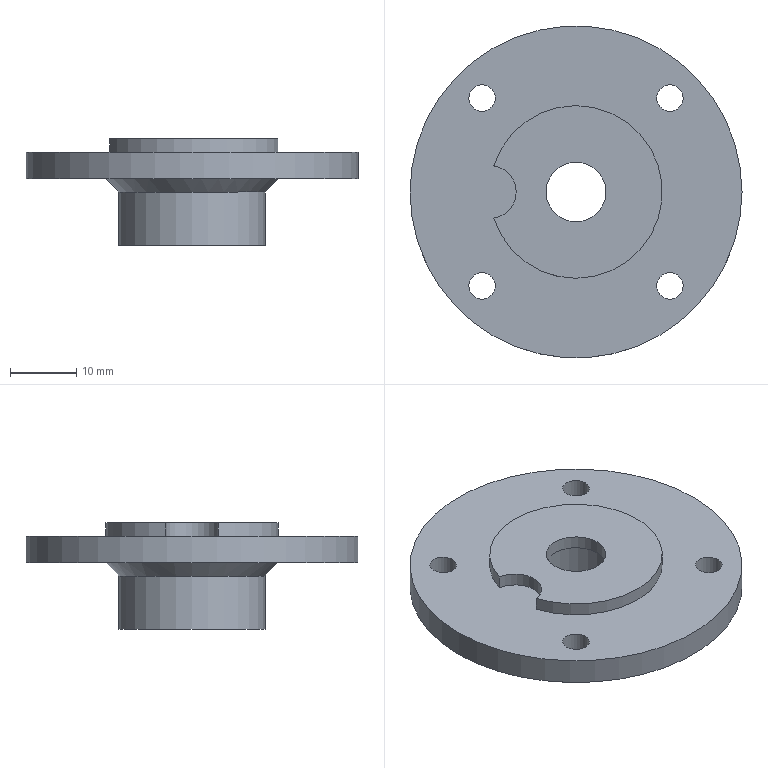Component | NX | 07__27_2 | 1 solid | 16 faces | box 50 x 50 x 16 mm | volume 10905 mm3 | cylinder 10 | plane 5 | cone 1 | commonest cylinder face diameters 4 x4 9 x1 12 x1 22 x1 50 x1 26 x1 8 x1
STEP:
#1=CARTESIAN_POINT('',(0.,0.,0.));
#2=DIRECTION('',(0.,0.,1.));
#3=DIRECTION('',(1.,0.,0.));
#4=AXIS2_PLACEMENT_3D('',#1,#2,#3);
#5=CARTESIAN_POINT('',(111.522,109.608,186.432));
#6=VERTEX_POINT('',#5);
#7=CARTESIAN_POINT('',(116.022,109.608,186.432));
#8=DIRECTION('',(0.,0.,-1.));
#9=DIRECTION('',(-1.,0.,-0.));
#10=AXIS2_PLACEMENT_3D('',#7,#8,#9);
#11=CIRCLE('',#10,4.5);
#12=CARTESIAN_POINT('',(116.022,109.608,188.432));
#13=DIRECTION('',(0.,0.,-1.));
#14=DIRECTION('',(-1.,0.,-0.));
#15=AXIS2_PLACEMENT_3D('',#12,#13,#14);
#16=CYLINDRICAL_SURFACE('',#15,4.5);
#17=CARTESIAN_POINT('',(0.,2.));
#18=DIRECTION('',(1.,0.));
#19=VECTOR('',#18,1.);
#20=LINE('',#17,#19);
#21=(GEOMETRIC_REPRESENTATION_CONTEXT(2)PARAMETRIC_REPRESENTATION_CONTEXT()REPRESENTATION_CONTEXT('',''));
#22=DEFINITIONAL_REPRESENTATION('',(#20),#21);
#23=PCURVE('',#16,#22);
#24=CARTESIAN_POINT('',(111.522,109.608,186.432));
#25=DIRECTION('',(0.,0.,-1.));
#26=DIRECTION('',(-1.,0.,-0.));
#27=AXIS2_PLACEMENT_3D('',#24,#25,#26);
#28=PLANE('',#27);
#29=CARTESIAN_POINT('',(-4.5,0.));
#30=DIRECTION('',(1.,0.));
#31=AXIS2_PLACEMENT_2D('',#29,#30);
#32=CIRCLE('',#31,4.5);
#33=(GEOMETRIC_REPRESENTATION_CONTEXT(2)PARAMETRIC_REPRESENTATION_CONTEXT()REPRESENTATION_CONTEXT('',''));
#34=DEFINITIONAL_REPRESENTATION('',(#32),#33);
#35=PCURVE('',#28,#34);
#36=SURFACE_CURVE('',#11,(#23,#35),.PCURVE_S1.);
#37=EDGE_CURVE('',#6,#6,#36,.T.);
#38=ORIENTED_EDGE('',*,*,#37,.F.);
#39=CARTESIAN_POINT('',(111.522,109.608,188.432));
#40=VERTEX_POINT('',#39);
#41=CARTESIAN_POINT('',(111.522,109.608,188.432));
#42=CARTESIAN_POINT('',(111.522,109.608,186.432));
#43=B_SPLINE_CURVE_WITH_KNOTS('',1,(#41,#42),.UNSPECIFIED.,.F.,.F.,(2,2),(0.,2.),.PIECEWISE_BEZIER_KNOTS.);
#44=CARTESIAN_POINT('',(0.,0.));
#45=DIRECTION('',(0.,1.));
#46=VECTOR('',#45,1.);
#47=LINE('',#44,#46);
#48=(GEOMETRIC_REPRESENTATION_CONTEXT(2)PARAMETRIC_REPRESENTATION_CONTEXT()REPRESENTATION_CONTEXT('',''));
#49=DEFINITIONAL_REPRESENTATION('',(#47),#48);
#50=PCURVE('',#16,#49);
#51=CARTESIAN_POINT('',(6.283,0.));
#52=DIRECTION('',(0.,1.));
#53=VECTOR('',#52,1.);
#54=LINE('',#51,#53);
#55=(GEOMETRIC_REPRESENTATION_CONTEXT(2)PARAMETRIC_REPRESENTATION_CONTEXT()REPRESENTATION_CONTEXT('',''));
#56=DEFINITIONAL_REPRESENTATION('',(#54),#55);
#57=PCURVE('',#16,#56);
#58=SEAM_CURVE('',#43,(#50,#57),.PCURVE_S1.);
#59=EDGE_CURVE('',#40,#6,#58,.T.);
#60=ORIENTED_EDGE('',*,*,#59,.F.);
#61=CARTESIAN_POINT('',(116.022,109.608,188.432));
#62=DIRECTION('',(0.,0.,-1.));
#63=DIRECTION('',(-1.,0.,-0.));
#64=AXIS2_PLACEMENT_3D('',#61,#62,#63);
#65=CIRCLE('',#64,4.5);
#66=CARTESIAN_POINT('',(0.,0.));
#67=DIRECTION('',(1.,0.));
#68=VECTOR('',#67,1.);
#69=LINE('',#66,#68);
#70=(GEOMETRIC_REPRESENTATION_CONTEXT(2)PARAMETRIC_REPRESENTATION_CONTEXT()REPRESENTATION_CONTEXT('',''));
#71=DEFINITIONAL_REPRESENTATION('',(#69),#70);
#72=PCURVE('',#16,#71);
#73=CARTESIAN_POINT('',(103.022,109.608,188.432));
#74=DIRECTION('',(-0.,0.,1.));
#75=DIRECTION('',(1.,0.,0.));
#76=AXIS2_PLACEMENT_3D('',#73,#74,#75);
#77=PLANE('',#76);
#78=CARTESIAN_POINT('',(8.5,0.));
#79=CARTESIAN_POINT('',(8.5,7.794));
#80=CARTESIAN_POINT('',(15.25,3.897));
#81=CARTESIAN_POINT('',(22.,0.));
#82=CARTESIAN_POINT('',(15.25,-3.897));
#83=CARTESIAN_POINT('',(8.5,-7.794));
#84=CARTESIAN_POINT('',(8.5,0.));
#85=(BOUNDED_CURVE()B_SPLINE_CURVE(2,(#78,#79,#80,#81,#82,#83,#84),.UNSPECIFIED.,.T.,.F.)B_SPLINE_CURVE_WITH_KNOTS((1,2,2,2,2,1),(-2.094,0.,2.094,4.189,6.283,8.378),.UNSPECIFIED.)CURVE()GEOMETRIC_REPRESENTATION_ITEM()RATIONAL_B_SPLINE_CURVE((1.,0.5,1.,0.5,1.,0.5,1.))REPRESENTATION_ITEM(''));
#86=(GEOMETRIC_REPRESENTATION_CONTEXT(2)PARAMETRIC_REPRESENTATION_CONTEXT()REPRESENTATION_CONTEXT('',''));
#87=DEFINITIONAL_REPRESENTATION('',(#85),#86);
#88=PCURVE('',#77,#87);
#89=SURFACE_CURVE('',#65,(#72,#88),.PCURVE_S1.);
#90=EDGE_CURVE('',#40,#40,#89,.T.);
#91=ORIENTED_EDGE('',*,*,#90,.T.);
#92=ORIENTED_EDGE('',*,*,#59,.T.);
#93=EDGE_LOOP('',(#38,#60,#91,#92));
#94=FACE_BOUND('',#93,.F.);
#95=ADVANCED_FACE('',(#94),#16,.F.);
#96=CARTESIAN_POINT('',(110.022,109.608,186.432));
#97=VERTEX_POINT('',#96);
#98=CARTESIAN_POINT('',(116.022,109.608,186.432));
#99=DIRECTION('',(0.,0.,-1.));
#100=DIRECTION('',(-1.,0.,-0.));
#101=AXIS2_PLACEMENT_3D('',#98,#99,#100);
#102=CIRCLE('',#101,6.);
#103=CARTESIAN_POINT('',(-4.5,0.));
#104=DIRECTION('',(1.,0.));
#105=AXIS2_PLACEMENT_2D('',#103,#104);
#106=CIRCLE('',#105,6.);
#107=(GEOMETRIC_REPRESENTATION_CONTEXT(2)PARAMETRIC_REPRESENTATION_CONTEXT()REPRESENTATION_CONTEXT('',''));
#108=DEFINITIONAL_REPRESENTATION('',(#106),#107);
#109=PCURVE('',#28,#108);
#110=CARTESIAN_POINT('',(116.022,109.608,188.432));
#111=DIRECTION('',(0.,0.,-1.));
#112=DIRECTION('',(-1.,0.,-0.));
#113=AXIS2_PLACEMENT_3D('',#110,#111,#112);
#114=CYLINDRICAL_SURFACE('',#113,6.);
#115=CARTESIAN_POINT('',(0.,2.));
#116=DIRECTION('',(1.,0.));
#117=VECTOR('',#116,1.);
#118=LINE('',#115,#117);
#119=(GEOMETRIC_REPRESENTATION_CONTEXT(2)PARAMETRIC_REPRESENTATION_CONTEXT()REPRESENTATION_CONTEXT('',''));
#120=DEFINITIONAL_REPRESENTATION('',(#118),#119);
#121=PCURVE('',#114,#120);
#122=SURFACE_CURVE('',#102,(#109,#121),.PCURVE_S1.);
#123=EDGE_CURVE('',#97,#97,#122,.T.);
#124=ORIENTED_EDGE('',*,*,#123,.T.);
#125=EDGE_LOOP('',(#124));
#126=FACE_BOUND('',#125,.T.);
#127=ORIENTED_EDGE('',*,*,#37,.F.);
#128=EDGE_LOOP('',(#127));
#129=FACE_BOUND('',#128,.T.);
#130=ADVANCED_FACE('',(#126,#129),#28,.T.);
#131=CARTESIAN_POINT('',(110.022,109.608,172.432));
#132=VERTEX_POINT('',#131);
#133=CARTESIAN_POINT('',(116.022,109.608,172.432));
#134=DIRECTION('',(0.,0.,-1.));
#135=DIRECTION('',(-1.,0.,-0.));
#136=AXIS2_PLACEMENT_3D('',#133,#134,#135);
#137=CIRCLE('',#136,6.);
#138=CARTESIAN_POINT('',(0.,16.));
#139=DIRECTION('',(1.,0.));
#140=VECTOR('',#139,1.);
#141=LINE('',#138,#140);
#142=(GEOMETRIC_REPRESENTATION_CONTEXT(2)PARAMETRIC_REPRESENTATION_CONTEXT()REPRESENTATION_CONTEXT('',''));
#143=DEFINITIONAL_REPRESENTATION('',(#141),#142);
#144=PCURVE('',#114,#143);
#145=CARTESIAN_POINT('',(110.022,109.608,172.432));
#146=DIRECTION('',(0.,0.,-1.));
#147=DIRECTION('',(-1.,0.,-0.));
#148=AXIS2_PLACEMENT_3D('',#145,#146,#147);
#149=PLANE('',#148);
#150=CARTESIAN_POINT('',(-6.,0.));
#151=DIRECTION('',(1.,0.));
#152=AXIS2_PLACEMENT_2D('',#150,#151);
#153=CIRCLE('',#152,6.);
#154=(GEOMETRIC_REPRESENTATION_CONTEXT(2)PARAMETRIC_REPRESENTATION_CONTEXT()REPRESENTATION_CONTEXT('',''));
#155=DEFINITIONAL_REPRESENTATION('',(#153),#154);
#156=PCURVE('',#149,#155);
#157=SURFACE_CURVE('',#137,(#144,#156),.PCURVE_S1.);
#158=EDGE_CURVE('',#132,#132,#157,.T.);
#159=ORIENTED_EDGE('',*,*,#158,.F.);
#160=CARTESIAN_POINT('',(110.022,109.608,186.432));
#161=CARTESIAN_POINT('',(110.022,109.608,172.432));
#162=B_SPLINE_CURVE_WITH_KNOTS('',1,(#160,#161),.UNSPECIFIED.,.F.,.F.,(2,2),(2.,16.),.PIECEWISE_BEZIER_KNOTS.);
#163=CARTESIAN_POINT('',(0.,0.));
#164=DIRECTION('',(0.,1.));
#165=VECTOR('',#164,1.);
#166=LINE('',#163,#165);
#167=(GEOMETRIC_REPRESENTATION_CONTEXT(2)PARAMETRIC_REPRESENTATION_CONTEXT()REPRESENTATION_CONTEXT('',''));
#168=DEFINITIONAL_REPRESENTATION('',(#166),#167);
#169=PCURVE('',#114,#168);
#170=CARTESIAN_POINT('',(6.283,0.));
#171=DIRECTION('',(0.,1.));
#172=VECTOR('',#171,1.);
#173=LINE('',#170,#172);
#174=(GEOMETRIC_REPRESENTATION_CONTEXT(2)PARAMETRIC_REPRESENTATION_CONTEXT()REPRESENTATION_CONTEXT('',''));
#175=DEFINITIONAL_REPRESENTATION('',(#173),#174);
#176=PCURVE('',#114,#175);
#177=SEAM_CURVE('',#162,(#169,#176),.PCURVE_S1.);
#178=EDGE_CURVE('',#97,#132,#177,.T.);
#179=ORIENTED_EDGE('',*,*,#178,.F.);
#180=ORIENTED_EDGE('',*,*,#123,.T.);
#181=ORIENTED_EDGE('',*,*,#178,.T.);
#182=EDGE_LOOP('',(#159,#179,#180,#181));
#183=FACE_BOUND('',#182,.F.);
#184=ADVANCED_FACE('',(#183),#114,.F.);
#185=CARTESIAN_POINT('',(105.022,109.608,172.432));
#186=VERTEX_POINT('',#185);
#187=CARTESIAN_POINT('',(116.022,109.608,172.432));
#188=DIRECTION('',(0.,0.,-1.));
#189=DIRECTION('',(-1.,0.,-0.));
#190=AXIS2_PLACEMENT_3D('',#187,#188,#189);
#191=CIRCLE('',#190,11.);
#192=CARTESIAN_POINT('',(-6.,0.));
#193=DIRECTION('',(1.,0.));
#194=AXIS2_PLACEMENT_2D('',#192,#193);
#195=CIRCLE('',#194,11.);
#196=(GEOMETRIC_REPRESENTATION_CONTEXT(2)PARAMETRIC_REPRESENTATION_CONTEXT()REPRESENTATION_CONTEXT('',''));
#197=DEFINITIONAL_REPRESENTATION('',(#195),#196);
#198=PCURVE('',#149,#197);
#199=CARTESIAN_POINT('',(116.022,109.608,188.432));
#200=DIRECTION('',(0.,0.,-1.));
#201=DIRECTION('',(-1.,0.,-0.));
#202=AXIS2_PLACEMENT_3D('',#199,#200,#201);
#203=CYLINDRICAL_SURFACE('',#202,11.);
#204=CARTESIAN_POINT('',(0.,16.));
#205=DIRECTION('',(1.,0.));
#206=VECTOR('',#205,1.);
#207=LINE('',#204,#206);
#208=(GEOMETRIC_REPRESENTATION_CONTEXT(2)PARAMETRIC_REPRESENTATION_CONTEXT()REPRESENTATION_CONTEXT('',''));
#209=DEFINITIONAL_REPRESENTATION('',(#207),#208);
#210=PCURVE('',#203,#209);
#211=SURFACE_CURVE('',#191,(#198,#210),.PCURVE_S1.);
#212=EDGE_CURVE('',#186,#186,#211,.T.);
#213=ORIENTED_EDGE('',*,*,#212,.T.);
#214=EDGE_LOOP('',(#213));
#215=FACE_BOUND('',#214,.T.);
#216=ORIENTED_EDGE('',*,*,#158,.F.);
#217=EDGE_LOOP('',(#216));
#218=FACE_BOUND('',#217,.T.);
#219=ADVANCED_FACE('',(#215,#218),#149,.T.);
#220=CARTESIAN_POINT('',(105.022,109.608,180.432));
#221=VERTEX_POINT('',#220);
#222=CARTESIAN_POINT('',(116.022,109.608,180.432));
#223=DIRECTION('',(0.,0.,-1.));
#224=DIRECTION('',(-1.,0.,-0.));
#225=AXIS2_PLACEMENT_3D('',#222,#223,#224);
#226=CIRCLE('',#225,11.);
#227=CARTESIAN_POINT('',(0.,8.));
#228=DIRECTION('',(1.,0.));
#229=VECTOR('',#228,1.);
#230=LINE('',#227,#229);
#231=(GEOMETRIC_REPRESENTATION_CONTEXT(2)PARAMETRIC_REPRESENTATION_CONTEXT()REPRESENTATION_CONTEXT('',''));
#232=DEFINITIONAL_REPRESENTATION('',(#230),#231);
#233=PCURVE('',#203,#232);
#234=CARTESIAN_POINT('',(116.022,109.608,180.432));
#235=DIRECTION('',(-0.,0.,1.));
#236=DIRECTION('',(1.,0.,0.));
#237=AXIS2_PLACEMENT_3D('',#234,#235,#236);
#238=CONICAL_SURFACE('',#237,11.,0.7854);
#239=CARTESIAN_POINT('',(9.425,0.));
#240=DIRECTION('',(-1.,0.));
#241=VECTOR('',#240,1.);
#242=LINE('',#239,#241);
#243=(GEOMETRIC_REPRESENTATION_CONTEXT(2)PARAMETRIC_REPRESENTATION_CONTEXT()REPRESENTATION_CONTEXT('',''));
#244=DEFINITIONAL_REPRESENTATION('',(#242),#243);
#245=PCURVE('',#238,#244);
#246=SURFACE_CURVE('',#226,(#233,#245),.PCURVE_S1.);
#247=EDGE_CURVE('',#221,#221,#246,.T.);
#248=ORIENTED_EDGE('',*,*,#247,.T.);
#249=CARTESIAN_POINT('',(105.022,109.608,180.432));
#250=CARTESIAN_POINT('',(105.022,109.608,172.432));
#251=B_SPLINE_CURVE_WITH_KNOTS('',1,(#249,#250),.UNSPECIFIED.,.F.,.F.,(2,2),(8.,16.),.PIECEWISE_BEZIER_KNOTS.);
#252=CARTESIAN_POINT('',(6.283,0.));
#253=DIRECTION('',(0.,1.));
#254=VECTOR('',#253,1.);
#255=LINE('',#252,#254);
#256=(GEOMETRIC_REPRESENTATION_CONTEXT(2)PARAMETRIC_REPRESENTATION_CONTEXT()REPRESENTATION_CONTEXT('',''));
#257=DEFINITIONAL_REPRESENTATION('',(#255),#256);
#258=PCURVE('',#203,#257);
#259=CARTESIAN_POINT('',(0.,0.));
#260=DIRECTION('',(0.,1.));
#261=VECTOR('',#260,1.);
#262=LINE('',#259,#261);
#263=(GEOMETRIC_REPRESENTATION_CONTEXT(2)PARAMETRIC_REPRESENTATION_CONTEXT()REPRESENTATION_CONTEXT('',''));
#264=DEFINITIONAL_REPRESENTATION('',(#262),#263);
#265=PCURVE('',#203,#264);
#266=SEAM_CURVE('',#251,(#258,#265),.PCURVE_S1.);
#267=EDGE_CURVE('',#221,#186,#266,.T.);
#268=ORIENTED_EDGE('',*,*,#267,.T.);
#269=ORIENTED_EDGE('',*,*,#212,.F.);
#270=ORIENTED_EDGE('',*,*,#267,.F.);
#271=EDGE_LOOP('',(#248,#268,#269,#270));
#272=FACE_BOUND('',#271,.T.);
#273=ADVANCED_FACE('',(#272),#203,.T.);
#274=CARTESIAN_POINT('',(103.022,109.608,182.432));
#275=VERTEX_POINT('',#274);
#276=CARTESIAN_POINT('',(116.022,109.608,182.432));
#277=DIRECTION('',(-0.,0.,1.));
#278=DIRECTION('',(-1.,0.,-0.));
#279=AXIS2_PLACEMENT_3D('',#276,#277,#278);
#280=CIRCLE('',#279,13.);
#281=CARTESIAN_POINT('',(105.022,109.608,182.432));
#282=DIRECTION('',(0.,0.,-1.));
#283=DIRECTION('',(-1.,0.,-0.));
#284=AXIS2_PLACEMENT_3D('',#281,#282,#283);
#285=PLANE('',#284);
#286=CARTESIAN_POINT('',(2.,0.));
#287=CARTESIAN_POINT('',(2.,-22.517));
#288=CARTESIAN_POINT('',(-17.5,-11.258));
#289=CARTESIAN_POINT('',(-37.,-0.));
#290=CARTESIAN_POINT('',(-17.5,11.258));
#291=CARTESIAN_POINT('',(2.,22.517));
#292=CARTESIAN_POINT('',(2.,0.));
#293=(BOUNDED_CURVE()B_SPLINE_CURVE(2,(#286,#287,#288,#289,#290,#291,#292),.UNSPECIFIED.,.T.,.F.)B_SPLINE_CURVE_WITH_KNOTS((1,2,2,2,2,1),(-2.094,0.,2.094,4.189,6.283,8.378),.UNSPECIFIED.)CURVE()GEOMETRIC_REPRESENTATION_ITEM()RATIONAL_B_SPLINE_CURVE((1.,0.5,1.,0.5,1.,0.5,1.))REPRESENTATION_ITEM(''));
#294=(GEOMETRIC_REPRESENTATION_CONTEXT(2)PARAMETRIC_REPRESENTATION_CONTEXT()REPRESENTATION_CONTEXT('',''));
#295=DEFINITIONAL_REPRESENTATION('',(#293),#294);
#296=PCURVE('',#285,#295);
#297=CARTESIAN_POINT('',(3.142,2.));
#298=DIRECTION('',(1.,0.));
#299=VECTOR('',#298,1.);
#300=LINE('',#297,#299);
#301=(GEOMETRIC_REPRESENTATION_CONTEXT(2)PARAMETRIC_REPRESENTATION_CONTEXT()REPRESENTATION_CONTEXT('',''));
#302=DEFINITIONAL_REPRESENTATION('',(#300),#301);
#303=PCURVE('',#238,#302);
#304=SURFACE_CURVE('',#280,(#296,#303),.PCURVE_S1.);
#305=EDGE_CURVE('',#275,#275,#304,.T.);
#306=ORIENTED_EDGE('',*,*,#305,.T.);
#307=EDGE_LOOP('',(#306));
#308=FACE_BOUND('',#307,.T.);
#309=CARTESIAN_POINT('',(128.164,123.75,182.432));
#310=VERTEX_POINT('',#309);
#311=CARTESIAN_POINT('',(130.164,123.75,182.432));
#312=DIRECTION('',(0.,0.,-1.));
#313=DIRECTION('',(-1.,0.,-0.));
#314=AXIS2_PLACEMENT_3D('',#311,#312,#313);
#315=CIRCLE('',#314,2.);
#316=CARTESIAN_POINT('',(-25.142,14.142));
#317=DIRECTION('',(1.,0.));
#318=AXIS2_PLACEMENT_2D('',#316,#317);
#319=CIRCLE('',#318,2.);
#320=(GEOMETRIC_REPRESENTATION_CONTEXT(2)PARAMETRIC_REPRESENTATION_CONTEXT()REPRESENTATION_CONTEXT('',''));
#321=DEFINITIONAL_REPRESENTATION('',(#319),#320);
#322=PCURVE('',#285,#321);
#323=CARTESIAN_POINT('',(130.164,123.75,170.132));
#324=DIRECTION('',(0.,0.,1.));
#325=DIRECTION('',(0.,1.,0.));
#326=AXIS2_PLACEMENT_3D('',#323,#324,#325);
#327=CYLINDRICAL_SURFACE('',#326,2.);
#328=CARTESIAN_POINT('',(7.854,12.3));
#329=DIRECTION('',(-1.,0.));
#330=VECTOR('',#329,1.);
#331=LINE('',#328,#330);
#332=(GEOMETRIC_REPRESENTATION_CONTEXT(2)PARAMETRIC_REPRESENTATION_CONTEXT()REPRESENTATION_CONTEXT('',''));
#333=DEFINITIONAL_REPRESENTATION('',(#331),#332);
#334=PCURVE('',#327,#333);
#335=SURFACE_CURVE('',#315,(#322,#334),.PCURVE_S1.);
#336=EDGE_CURVE('',#310,#310,#335,.T.);
#337=ORIENTED_EDGE('',*,*,#336,.F.);
#338=EDGE_LOOP('',(#337));
#339=FACE_BOUND('',#338,.T.);
#340=CARTESIAN_POINT('',(99.88,95.466,182.432));
#341=VERTEX_POINT('',#340);
#342=CARTESIAN_POINT('',(101.88,95.466,182.432));
#343=DIRECTION('',(0.,0.,-1.));
#344=DIRECTION('',(-1.,0.,-0.));
#345=AXIS2_PLACEMENT_3D('',#342,#343,#344);
#346=CIRCLE('',#345,2.);
#347=CARTESIAN_POINT('',(3.142,-14.142));
#348=DIRECTION('',(1.,0.));
#349=AXIS2_PLACEMENT_2D('',#347,#348);
#350=CIRCLE('',#349,2.);
#351=(GEOMETRIC_REPRESENTATION_CONTEXT(2)PARAMETRIC_REPRESENTATION_CONTEXT()REPRESENTATION_CONTEXT('',''));
#352=DEFINITIONAL_REPRESENTATION('',(#350),#351);
#353=PCURVE('',#285,#352);
#354=CARTESIAN_POINT('',(101.88,95.466,170.132));
#355=DIRECTION('',(0.,0.,1.));
#356=DIRECTION('',(0.,1.,0.));
#357=AXIS2_PLACEMENT_3D('',#354,#355,#356);
#358=CYLINDRICAL_SURFACE('',#357,2.);
#359=CARTESIAN_POINT('',(7.854,12.3));
#360=DIRECTION('',(-1.,0.));
#361=VECTOR('',#360,1.);
#362=LINE('',#359,#361);
#363=(GEOMETRIC_REPRESENTATION_CONTEXT(2)PARAMETRIC_REPRESENTATION_CONTEXT()REPRESENTATION_CONTEXT('',''));
#364=DEFINITIONAL_REPRESENTATION('',(#362),#363);
#365=PCURVE('',#358,#364);
#366=SURFACE_CURVE('',#346,(#353,#365),.PCURVE_S1.);
#367=EDGE_CURVE('',#341,#341,#366,.T.);
#368=ORIENTED_EDGE('',*,*,#367,.F.);
#369=EDGE_LOOP('',(#368));
#370=FACE_BOUND('',#369,.T.);
#371=CARTESIAN_POINT('',(128.164,95.466,182.432));
#372=VERTEX_POINT('',#371);
#373=CARTESIAN_POINT('',(130.164,95.466,182.432));
#374=DIRECTION('',(0.,0.,-1.));
#375=DIRECTION('',(-1.,0.,-0.));
#376=AXIS2_PLACEMENT_3D('',#373,#374,#375);
#377=CIRCLE('',#376,2.);
#378=CARTESIAN_POINT('',(-25.142,-14.142));
#379=DIRECTION('',(1.,0.));
#380=AXIS2_PLACEMENT_2D('',#378,#379);
#381=CIRCLE('',#380,2.);
#382=(GEOMETRIC_REPRESENTATION_CONTEXT(2)PARAMETRIC_REPRESENTATION_CONTEXT()REPRESENTATION_CONTEXT('',''));
#383=DEFINITIONAL_REPRESENTATION('',(#381),#382);
#384=PCURVE('',#285,#383);
#385=CARTESIAN_POINT('',(130.164,95.466,170.132));
#386=DIRECTION('',(0.,0.,1.));
#387=DIRECTION('',(0.,1.,0.));
#388=AXIS2_PLACEMENT_3D('',#385,#386,#387);
#389=CYLINDRICAL_SURFACE('',#388,2.);
#390=CARTESIAN_POINT('',(7.854,12.3));
#391=DIRECTION('',(-1.,0.));
#392=VECTOR('',#391,1.);
#393=LINE('',#390,#392);
#394=(GEOMETRIC_REPRESENTATION_CONTEXT(2)PARAMETRIC_REPRESENTATION_CONTEXT()REPRESENTATION_CONTEXT('',''));
#395=DEFINITIONAL_REPRESENTATION('',(#393),#394);
#396=PCURVE('',#389,#395);
#397=SURFACE_CURVE('',#377,(#384,#396),.PCURVE_S1.);
#398=EDGE_CURVE('',#372,#372,#397,.T.);
#399=ORIENTED_EDGE('',*,*,#398,.F.);
#400=EDGE_LOOP('',(#399));
#401=FACE_BOUND('',#400,.T.);
#402=CARTESIAN_POINT('',(99.88,123.75,182.432));
#403=VERTEX_POINT('',#402);
#404=CARTESIAN_POINT('',(101.88,123.75,182.432));
#405=DIRECTION('',(0.,0.,-1.));
#406=DIRECTION('',(-1.,0.,-0.));
#407=AXIS2_PLACEMENT_3D('',#404,#405,#406);
#408=CIRCLE('',#407,2.);
#409=CARTESIAN_POINT('',(3.142,14.142));
#410=DIRECTION('',(1.,0.));
#411=AXIS2_PLACEMENT_2D('',#409,#410);
#412=CIRCLE('',#411,2.);
#413=(GEOMETRIC_REPRESENTATION_CONTEXT(2)PARAMETRIC_REPRESENTATION_CONTEXT()REPRESENTATION_CONTEXT('',''));
#414=DEFINITIONAL_REPRESENTATION('',(#412),#413);
#415=PCURVE('',#285,#414);
#416=CARTESIAN_POINT('',(101.88,123.75,170.132));
#417=DIRECTION('',(0.,0.,1.));
#418=DIRECTION('',(0.,1.,0.));
#419=AXIS2_PLACEMENT_3D('',#416,#417,#418);
#420=CYLINDRICAL_SURFACE('',#419,2.);
#421=CARTESIAN_POINT('',(7.854,12.3));
#422=DIRECTION('',(-1.,0.));
#423=VECTOR('',#422,1.);
#424=LINE('',#421,#423);
#425=(GEOMETRIC_REPRESENTATION_CONTEXT(2)PARAMETRIC_REPRESENTATION_CONTEXT()REPRESENTATION_CONTEXT('',''));
#426=DEFINITIONAL_REPRESENTATION('',(#424),#425);
#427=PCURVE('',#420,#426);
#428=SURFACE_CURVE('',#408,(#415,#427),.PCURVE_S1.);
#429=EDGE_CURVE('',#403,#403,#428,.T.);
#430=ORIENTED_EDGE('',*,*,#429,.F.);
#431=EDGE_LOOP('',(#430));
#432=FACE_BOUND('',#431,.T.);
#433=CARTESIAN_POINT('',(91.022,109.608,182.432));
#434=VERTEX_POINT('',#433);
#435=CARTESIAN_POINT('',(116.022,109.608,182.432));
#436=DIRECTION('',(0.,0.,-1.));
#437=DIRECTION('',(-1.,0.,-0.));
#438=AXIS2_PLACEMENT_3D('',#435,#436,#437);
#439=CIRCLE('',#438,25.);
#440=CARTESIAN_POINT('',(-11.,0.));
#441=DIRECTION('',(1.,0.));
#442=AXIS2_PLACEMENT_2D('',#440,#441);
#443=CIRCLE('',#442,25.);
#444=(GEOMETRIC_REPRESENTATION_CONTEXT(2)PARAMETRIC_REPRESENTATION_CONTEXT()REPRESENTATION_CONTEXT('',''));
#445=DEFINITIONAL_REPRESENTATION('',(#443),#444);
#446=PCURVE('',#285,#445);
#447=CARTESIAN_POINT('',(116.022,109.608,188.432));
#448=DIRECTION('',(0.,0.,-1.));
#449=DIRECTION('',(-1.,0.,-0.));
#450=AXIS2_PLACEMENT_3D('',#447,#448,#449);
#451=CYLINDRICAL_SURFACE('',#450,25.);
#452=CARTESIAN_POINT('',(0.,6.));
#453=DIRECTION('',(1.,0.));
#454=VECTOR('',#453,1.);
#455=LINE('',#452,#454);
#456=(GEOMETRIC_REPRESENTATION_CONTEXT(2)PARAMETRIC_REPRESENTATION_CONTEXT()REPRESENTATION_CONTEXT('',''));
#457=DEFINITIONAL_REPRESENTATION('',(#455),#456);
#458=PCURVE('',#451,#457);
#459=SURFACE_CURVE('',#439,(#446,#458),.PCURVE_S1.);
#460=EDGE_CURVE('',#434,#434,#459,.T.);
#461=ORIENTED_EDGE('',*,*,#460,.T.);
#462=EDGE_LOOP('',(#461));
#463=FACE_BOUND('',#462,.T.);
#464=ADVANCED_FACE('',(#308,#339,#370,#401,#432,#463),#285,.T.);
#465=CARTESIAN_POINT('',(91.022,109.608,186.432));
#466=VERTEX_POINT('',#465);
#467=CARTESIAN_POINT('',(116.022,109.608,186.432));
#468=DIRECTION('',(0.,0.,-1.));
#469=DIRECTION('',(-1.,0.,-0.));
#470=AXIS2_PLACEMENT_3D('',#467,#468,#469);
#471=CIRCLE('',#470,25.);
#472=CARTESIAN_POINT('',(0.,2.));
#473=DIRECTION('',(1.,0.));
#474=VECTOR('',#473,1.);
#475=LINE('',#472,#474);
#476=(GEOMETRIC_REPRESENTATION_CONTEXT(2)PARAMETRIC_REPRESENTATION_CONTEXT()REPRESENTATION_CONTEXT('',''));
#477=DEFINITIONAL_REPRESENTATION('',(#475),#476);
#478=PCURVE('',#451,#477);
#479=CARTESIAN_POINT('',(91.022,109.608,186.432));
#480=DIRECTION('',(-0.,0.,1.));
#481=DIRECTION('',(1.,0.,0.));
#482=AXIS2_PLACEMENT_3D('',#479,#480,#481);
#483=PLANE('',#482);
#484=CARTESIAN_POINT('',(0.,0.));
#485=CARTESIAN_POINT('',(0.,43.301));
#486=CARTESIAN_POINT('',(37.5,21.651));
#487=CARTESIAN_POINT('',(75.,0.));
#488=CARTESIAN_POINT('',(37.5,-21.651));
#489=CARTESIAN_POINT('',(0.,-43.301));
#490=CARTESIAN_POINT('',(0.,0.));
#491=(BOUNDED_CURVE()B_SPLINE_CURVE(2,(#484,#485,#486,#487,#488,#489,#490),.UNSPECIFIED.,.T.,.F.)B_SPLINE_CURVE_WITH_KNOTS((1,2,2,2,2,1),(-2.094,0.,2.094,4.189,6.283,8.378),.UNSPECIFIED.)CURVE()GEOMETRIC_REPRESENTATION_ITEM()RATIONAL_B_SPLINE_CURVE((1.,0.5,1.,0.5,1.,0.5,1.))REPRESENTATION_ITEM(''));
#492=(GEOMETRIC_REPRESENTATION_CONTEXT(2)PARAMETRIC_REPRESENTATION_CONTEXT()REPRESENTATION_CONTEXT('',''));
#493=DEFINITIONAL_REPRESENTATION('',(#491),#492);
#494=PCURVE('',#483,#493);
#495=SURFACE_CURVE('',#471,(#478,#494),.PCURVE_S1.);
#496=EDGE_CURVE('',#466,#466,#495,.T.);
#497=ORIENTED_EDGE('',*,*,#496,.T.);
#498=CARTESIAN_POINT('',(91.022,109.608,186.432));
#499=CARTESIAN_POINT('',(91.022,109.608,182.432));
#500=B_SPLINE_CURVE_WITH_KNOTS('',1,(#498,#499),.UNSPECIFIED.,.F.,.F.,(2,2),(2.,6.),.PIECEWISE_BEZIER_KNOTS.);
#501=CARTESIAN_POINT('',(6.283,0.));
#502=DIRECTION('',(0.,1.));
#503=VECTOR('',#502,1.);
#504=LINE('',#501,#503);
#505=(GEOMETRIC_REPRESENTATION_CONTEXT(2)PARAMETRIC_REPRESENTATION_CONTEXT()REPRESENTATION_CONTEXT('',''));
#506=DEFINITIONAL_REPRESENTATION('',(#504),#505);
#507=PCURVE('',#451,#506);
#508=CARTESIAN_POINT('',(0.,0.));
#509=DIRECTION('',(0.,1.));
#510=VECTOR('',#509,1.);
#511=LINE('',#508,#510);
#512=(GEOMETRIC_REPRESENTATION_CONTEXT(2)PARAMETRIC_REPRESENTATION_CONTEXT()REPRESENTATION_CONTEXT('',''));
#513=DEFINITIONAL_REPRESENTATION('',(#511),#512);
#514=PCURVE('',#451,#513);
#515=SEAM_CURVE('',#500,(#507,#514),.PCURVE_S1.);
#516=EDGE_CURVE('',#466,#434,#515,.T.);
#517=ORIENTED_EDGE('',*,*,#516,.T.);
#518=ORIENTED_EDGE('',*,*,#460,.F.);
#519=ORIENTED_EDGE('',*,*,#516,.F.);
#520=EDGE_LOOP('',(#497,#517,#518,#519));
#521=FACE_BOUND('',#520,.T.);
#522=ADVANCED_FACE('',(#521),#451,.T.);
#523=CARTESIAN_POINT('',(103.638,113.56,186.432));
#524=VERTEX_POINT('',#523);
#525=CARTESIAN_POINT('',(103.638,105.656,186.432));
#526=VERTEX_POINT('',#525);
#527=CARTESIAN_POINT('',(116.022,109.608,186.432));
#528=DIRECTION('',(0.,0.,-1.));
#529=DIRECTION('',(-1.,0.,-0.));
#530=AXIS2_PLACEMENT_3D('',#527,#528,#529);
#531=CIRCLE('',#530,13.);
#532=CARTESIAN_POINT('',(12.,0.));
#533=CARTESIAN_POINT('',(12.,22.517));
#534=CARTESIAN_POINT('',(31.5,11.258));
#535=CARTESIAN_POINT('',(51.,0.));
#536=CARTESIAN_POINT('',(31.5,-11.258));
#537=CARTESIAN_POINT('',(12.,-22.517));
#538=CARTESIAN_POINT('',(12.,0.));
#539=(BOUNDED_CURVE()B_SPLINE_CURVE(2,(#532,#533,#534,#535,#536,#537,#538),.UNSPECIFIED.,.T.,.F.)B_SPLINE_CURVE_WITH_KNOTS((1,2,2,2,2,1),(-2.094,0.,2.094,4.189,6.283,8.378),.UNSPECIFIED.)CURVE()GEOMETRIC_REPRESENTATION_ITEM()RATIONAL_B_SPLINE_CURVE((1.,0.5,1.,0.5,1.,0.5,1.))REPRESENTATION_ITEM(''));
#540=(GEOMETRIC_REPRESENTATION_CONTEXT(2)PARAMETRIC_REPRESENTATION_CONTEXT()REPRESENTATION_CONTEXT('',''));
#541=DEFINITIONAL_REPRESENTATION('',(#539),#540);
#542=PCURVE('',#483,#541);
#543=CARTESIAN_POINT('',(116.022,109.608,188.432));
#544=DIRECTION('',(0.,0.,-1.));
#545=DIRECTION('',(-1.,0.,-0.));
#546=AXIS2_PLACEMENT_3D('',#543,#544,#545);
#547=CYLINDRICAL_SURFACE('',#546,13.);
#548=CARTESIAN_POINT('',(0.,2.));
#549=DIRECTION('',(1.,0.));
#550=VECTOR('',#549,1.);
#551=LINE('',#548,#550);
#552=(GEOMETRIC_REPRESENTATION_CONTEXT(2)PARAMETRIC_REPRESENTATION_CONTEXT()REPRESENTATION_CONTEXT('',''));
#553=DEFINITIONAL_REPRESENTATION('',(#551),#552);
#554=PCURVE('',#547,#553);
#555=SURFACE_CURVE('',#531,(#542,#554),.PCURVE_S1.);
#556=EDGE_CURVE('',#524,#526,#555,.T.);
#557=ORIENTED_EDGE('',*,*,#556,.T.);
#558=CARTESIAN_POINT('',(103.022,109.608,186.432));
#559=DIRECTION('',(0.,0.,1.));
#560=DIRECTION('',(0.,1.,0.));
#561=AXIS2_PLACEMENT_3D('',#558,#559,#560);
#562=CIRCLE('',#561,4.);
#563=CARTESIAN_POINT('',(12.,0.));
#564=DIRECTION('',(0.,1.));
#565=AXIS2_PLACEMENT_2D('',#563,#564);
#566=CIRCLE('',#565,4.);
#567=(GEOMETRIC_REPRESENTATION_CONTEXT(2)PARAMETRIC_REPRESENTATION_CONTEXT()REPRESENTATION_CONTEXT('',''));
#568=DEFINITIONAL_REPRESENTATION('',(#566),#567);
#569=PCURVE('',#483,#568);
#570=CARTESIAN_POINT('',(103.022,109.608,186.432));
#571=DIRECTION('',(0.,0.,1.));
#572=DIRECTION('',(0.,1.,0.));
#573=AXIS2_PLACEMENT_3D('',#570,#571,#572);
#574=CYLINDRICAL_SURFACE('',#573,4.);
#575=CARTESIAN_POINT('',(0.,0.));
#576=DIRECTION('',(1.,0.));
#577=VECTOR('',#576,1.);
#578=LINE('',#575,#577);
#579=(GEOMETRIC_REPRESENTATION_CONTEXT(2)PARAMETRIC_REPRESENTATION_CONTEXT()REPRESENTATION_CONTEXT('',''));
#580=DEFINITIONAL_REPRESENTATION('',(#578),#579);
#581=PCURVE('',#574,#580);
#582=SURFACE_CURVE('',#562,(#569,#581),.PCURVE_S1.);
#583=EDGE_CURVE('',#526,#524,#582,.T.);
#584=ORIENTED_EDGE('',*,*,#583,.T.);
#585=EDGE_LOOP('',(#557,#584));
#586=FACE_BOUND('',#585,.T.);
#587=CARTESIAN_POINT('',(132.164,123.75,186.432));
#588=VERTEX_POINT('',#587);
#589=CARTESIAN_POINT('',(128.164,123.75,186.432));
#590=VERTEX_POINT('',#589);
#591=CARTESIAN_POINT('',(130.164,123.75,186.432));
#592=DIRECTION('',(-0.,0.,1.));
#593=DIRECTION('',(1.,0.,0.));
#594=AXIS2_PLACEMENT_3D('',#591,#592,#593);
#595=CIRCLE('',#594,2.);
#596=CARTESIAN_POINT('',(39.142,14.142));
#597=DIRECTION('',(1.,0.));
#598=AXIS2_PLACEMENT_2D('',#596,#597);
#599=CIRCLE('',#598,2.);
#600=(GEOMETRIC_REPRESENTATION_CONTEXT(2)PARAMETRIC_REPRESENTATION_CONTEXT()REPRESENTATION_CONTEXT('',''));
#601=DEFINITIONAL_REPRESENTATION('',(#599),#600);
#602=PCURVE('',#483,#601);
#603=CARTESIAN_POINT('',(4.712,16.3));
#604=DIRECTION('',(1.,0.));
#605=VECTOR('',#604,1.);
#606=LINE('',#603,#605);
#607=(GEOMETRIC_REPRESENTATION_CONTEXT(2)PARAMETRIC_REPRESENTATION_CONTEXT()REPRESENTATION_CONTEXT('',''));
#608=DEFINITIONAL_REPRESENTATION('',(#606),#607);
#609=PCURVE('',#327,#608);
#610=SURFACE_CURVE('',#595,(#602,#609),.PCURVE_S1.);
#611=EDGE_CURVE('',#588,#590,#610,.T.);
#612=ORIENTED_EDGE('',*,*,#611,.F.);
#613=CARTESIAN_POINT('',(130.164,123.75,186.432));
#614=DIRECTION('',(-0.,0.,1.));
#615=DIRECTION('',(1.,0.,0.));
#616=AXIS2_PLACEMENT_3D('',#613,#614,#615);
#617=CIRCLE('',#616,2.);
#618=CARTESIAN_POINT('',(39.142,14.142));
#619=DIRECTION('',(1.,0.));
#620=AXIS2_PLACEMENT_2D('',#618,#619);
#621=CIRCLE('',#620,2.);
#622=(GEOMETRIC_REPRESENTATION_CONTEXT(2)PARAMETRIC_REPRESENTATION_CONTEXT()REPRESENTATION_CONTEXT('',''));
#623=DEFINITIONAL_REPRESENTATION('',(#621),#622);
#624=PCURVE('',#483,#623);
#625=CARTESIAN_POINT('',(-1.571,16.3));
#626=DIRECTION('',(1.,0.));
#627=VECTOR('',#626,1.);
#628=LINE('',#625,#627);
#629=(GEOMETRIC_REPRESENTATION_CONTEXT(2)PARAMETRIC_REPRESENTATION_CONTEXT()REPRESENTATION_CONTEXT('',''));
#630=DEFINITIONAL_REPRESENTATION('',(#628),#629);
#631=PCURVE('',#327,#630);
#632=SURFACE_CURVE('',#617,(#624,#631),.PCURVE_S1.);
#633=EDGE_CURVE('',#590,#588,#632,.T.);
#634=ORIENTED_EDGE('',*,*,#633,.F.);
#635=EDGE_LOOP('',(#612,#634));
#636=FACE_BOUND('',#635,.T.);
#637=CARTESIAN_POINT('',(103.88,95.466,186.432));
#638=VERTEX_POINT('',#637);
#639=CARTESIAN_POINT('',(99.88,95.466,186.432));
#640=VERTEX_POINT('',#639);
#641=CARTESIAN_POINT('',(101.88,95.466,186.432));
#642=DIRECTION('',(-0.,0.,1.));
#643=DIRECTION('',(1.,0.,0.));
#644=AXIS2_PLACEMENT_3D('',#641,#642,#643);
#645=CIRCLE('',#644,2.);
#646=CARTESIAN_POINT('',(10.858,-14.142));
#647=DIRECTION('',(1.,0.));
#648=AXIS2_PLACEMENT_2D('',#646,#647);
#649=CIRCLE('',#648,2.);
#650=(GEOMETRIC_REPRESENTATION_CONTEXT(2)PARAMETRIC_REPRESENTATION_CONTEXT()REPRESENTATION_CONTEXT('',''));
#651=DEFINITIONAL_REPRESENTATION('',(#649),#650);
#652=PCURVE('',#483,#651);
#653=CARTESIAN_POINT('',(4.712,16.3));
#654=DIRECTION('',(1.,0.));
#655=VECTOR('',#654,1.);
#656=LINE('',#653,#655);
#657=(GEOMETRIC_REPRESENTATION_CONTEXT(2)PARAMETRIC_REPRESENTATION_CONTEXT()REPRESENTATION_CONTEXT('',''));
#658=DEFINITIONAL_REPRESENTATION('',(#656),#657);
#659=PCURVE('',#358,#658);
#660=SURFACE_CURVE('',#645,(#652,#659),.PCURVE_S1.);
#661=EDGE_CURVE('',#638,#640,#660,.T.);
#662=ORIENTED_EDGE('',*,*,#661,.F.);
#663=CARTESIAN_POINT('',(101.88,95.466,186.432));
#664=DIRECTION('',(-0.,0.,1.));
#665=DIRECTION('',(1.,0.,0.));
#666=AXIS2_PLACEMENT_3D('',#663,#664,#665);
#667=CIRCLE('',#666,2.);
#668=CARTESIAN_POINT('',(10.858,-14.142));
#669=DIRECTION('',(1.,0.));
#670=AXIS2_PLACEMENT_2D('',#668,#669);
#671=CIRCLE('',#670,2.);
#672=(GEOMETRIC_REPRESENTATION_CONTEXT(2)PARAMETRIC_REPRESENTATION_CONTEXT()REPRESENTATION_CONTEXT('',''));
#673=DEFINITIONAL_REPRESENTATION('',(#671),#672);
#674=PCURVE('',#483,#673);
#675=CARTESIAN_POINT('',(-1.571,16.3));
#676=DIRECTION('',(1.,0.));
#677=VECTOR('',#676,1.);
#678=LINE('',#675,#677);
#679=(GEOMETRIC_REPRESENTATION_CONTEXT(2)PARAMETRIC_REPRESENTATION_CONTEXT()REPRESENTATION_CONTEXT('',''));
#680=DEFINITIONAL_REPRESENTATION('',(#678),#679);
#681=PCURVE('',#358,#680);
#682=SURFACE_CURVE('',#667,(#674,#681),.PCURVE_S1.);
#683=EDGE_CURVE('',#640,#638,#682,.T.);
#684=ORIENTED_EDGE('',*,*,#683,.F.);
#685=EDGE_LOOP('',(#662,#684));
#686=FACE_BOUND('',#685,.T.);
#687=CARTESIAN_POINT('',(132.164,95.466,186.432));
#688=VERTEX_POINT('',#687);
#689=CARTESIAN_POINT('',(128.164,95.466,186.432));
#690=VERTEX_POINT('',#689);
#691=CARTESIAN_POINT('',(130.164,95.466,186.432));
#692=DIRECTION('',(-0.,0.,1.));
#693=DIRECTION('',(1.,0.,0.));
#694=AXIS2_PLACEMENT_3D('',#691,#692,#693);
#695=CIRCLE('',#694,2.);
#696=CARTESIAN_POINT('',(39.142,-14.142));
#697=DIRECTION('',(1.,0.));
#698=AXIS2_PLACEMENT_2D('',#696,#697);
#699=CIRCLE('',#698,2.);
#700=(GEOMETRIC_REPRESENTATION_CONTEXT(2)PARAMETRIC_REPRESENTATION_CONTEXT()REPRESENTATION_CONTEXT('',''));
#701=DEFINITIONAL_REPRESENTATION('',(#699),#700);
#702=PCURVE('',#483,#701);
#703=CARTESIAN_POINT('',(4.712,16.3));
#704=DIRECTION('',(1.,0.));
#705=VECTOR('',#704,1.);
#706=LINE('',#703,#705);
#707=(GEOMETRIC_REPRESENTATION_CONTEXT(2)PARAMETRIC_REPRESENTATION_CONTEXT()REPRESENTATION_CONTEXT('',''));
#708=DEFINITIONAL_REPRESENTATION('',(#706),#707);
#709=PCURVE('',#389,#708);
#710=SURFACE_CURVE('',#695,(#702,#709),.PCURVE_S1.);
#711=EDGE_CURVE('',#688,#690,#710,.T.);
#712=ORIENTED_EDGE('',*,*,#711,.F.);
#713=CARTESIAN_POINT('',(130.164,95.466,186.432));
#714=DIRECTION('',(-0.,0.,1.));
#715=DIRECTION('',(1.,0.,0.));
#716=AXIS2_PLACEMENT_3D('',#713,#714,#715);
#717=CIRCLE('',#716,2.);
#718=CARTESIAN_POINT('',(39.142,-14.142));
#719=DIRECTION('',(1.,0.));
#720=AXIS2_PLACEMENT_2D('',#718,#719);
#721=CIRCLE('',#720,2.);
#722=(GEOMETRIC_REPRESENTATION_CONTEXT(2)PARAMETRIC_REPRESENTATION_CONTEXT()REPRESENTATION_CONTEXT('',''));
#723=DEFINITIONAL_REPRESENTATION('',(#721),#722);
#724=PCURVE('',#483,#723);
#725=CARTESIAN_POINT('',(-1.571,16.3));
#726=DIRECTION('',(1.,0.));
#727=VECTOR('',#726,1.);
#728=LINE('',#725,#727);
#729=(GEOMETRIC_REPRESENTATION_CONTEXT(2)PARAMETRIC_REPRESENTATION_CONTEXT()REPRESENTATION_CONTEXT('',''));
#730=DEFINITIONAL_REPRESENTATION('',(#728),#729);
#731=PCURVE('',#389,#730);
#732=SURFACE_CURVE('',#717,(#724,#731),.PCURVE_S1.);
#733=EDGE_CURVE('',#690,#688,#732,.T.);
#734=ORIENTED_EDGE('',*,*,#733,.F.);
#735=EDGE_LOOP('',(#712,#734));
#736=FACE_BOUND('',#735,.T.);
#737=CARTESIAN_POINT('',(103.88,123.75,186.432));
#738=VERTEX_POINT('',#737);
#739=CARTESIAN_POINT('',(99.88,123.75,186.432));
#740=VERTEX_POINT('',#739);
#741=CARTESIAN_POINT('',(101.88,123.75,186.432));
#742=DIRECTION('',(-0.,0.,1.));
#743=DIRECTION('',(1.,0.,0.));
#744=AXIS2_PLACEMENT_3D('',#741,#742,#743);
#745=CIRCLE('',#744,2.);
#746=CARTESIAN_POINT('',(10.858,14.142));
#747=DIRECTION('',(1.,0.));
#748=AXIS2_PLACEMENT_2D('',#746,#747);
#749=CIRCLE('',#748,2.);
#750=(GEOMETRIC_REPRESENTATION_CONTEXT(2)PARAMETRIC_REPRESENTATION_CONTEXT()REPRESENTATION_CONTEXT('',''));
#751=DEFINITIONAL_REPRESENTATION('',(#749),#750);
#752=PCURVE('',#483,#751);
#753=CARTESIAN_POINT('',(4.712,16.3));
#754=DIRECTION('',(1.,0.));
#755=VECTOR('',#754,1.);
#756=LINE('',#753,#755);
#757=(GEOMETRIC_REPRESENTATION_CONTEXT(2)PARAMETRIC_REPRESENTATION_CONTEXT()REPRESENTATION_CONTEXT('',''));
#758=DEFINITIONAL_REPRESENTATION('',(#756),#757);
#759=PCURVE('',#420,#758);
#760=SURFACE_CURVE('',#745,(#752,#759),.PCURVE_S1.);
#761=EDGE_CURVE('',#738,#740,#760,.T.);
#762=ORIENTED_EDGE('',*,*,#761,.F.);
#763=CARTESIAN_POINT('',(101.88,123.75,186.432));
#764=DIRECTION('',(-0.,0.,1.));
#765=DIRECTION('',(1.,0.,0.));
#766=AXIS2_PLACEMENT_3D('',#763,#764,#765);
#767=CIRCLE('',#766,2.);
#768=CARTESIAN_POINT('',(10.858,14.142));
#769=DIRECTION('',(1.,0.));
#770=AXIS2_PLACEMENT_2D('',#768,#769);
#771=CIRCLE('',#770,2.);
#772=(GEOMETRIC_REPRESENTATION_CONTEXT(2)PARAMETRIC_REPRESENTATION_CONTEXT()REPRESENTATION_CONTEXT('',''));
#773=DEFINITIONAL_REPRESENTATION('',(#771),#772);
#774=PCURVE('',#483,#773);
#775=CARTESIAN_POINT('',(-1.571,16.3));
#776=DIRECTION('',(1.,0.));
#777=VECTOR('',#776,1.);
#778=LINE('',#775,#777);
#779=(GEOMETRIC_REPRESENTATION_CONTEXT(2)PARAMETRIC_REPRESENTATION_CONTEXT()REPRESENTATION_CONTEXT('',''));
#780=DEFINITIONAL_REPRESENTATION('',(#778),#779);
#781=PCURVE('',#420,#780);
#782=SURFACE_CURVE('',#767,(#774,#781),.PCURVE_S1.);
#783=EDGE_CURVE('',#740,#738,#782,.T.);
#784=ORIENTED_EDGE('',*,*,#783,.F.);
#785=EDGE_LOOP('',(#762,#784));
#786=FACE_BOUND('',#785,.T.);
#787=ORIENTED_EDGE('',*,*,#496,.F.);
#788=EDGE_LOOP('',(#787));
#789=FACE_BOUND('',#788,.T.);
#790=ADVANCED_FACE('',(#586,#636,#686,#736,#786,#789),#483,.T.);
#791=CARTESIAN_POINT('',(103.638,113.56,188.432));
#792=VERTEX_POINT('',#791);
#793=CARTESIAN_POINT('',(103.638,113.56,187.432));
#794=DIRECTION('',(0.,0.,-1.));
#795=VECTOR('',#794,1.);
#796=LINE('',#793,#795);
#797=CARTESIAN_POINT('',(0.3089,1.));
#798=DIRECTION('',(0.,1.));
#799=VECTOR('',#798,1.);
#800=LINE('',#797,#799);
#801=(GEOMETRIC_REPRESENTATION_CONTEXT(2)PARAMETRIC_REPRESENTATION_CONTEXT()REPRESENTATION_CONTEXT('',''));
#802=DEFINITIONAL_REPRESENTATION('',(#800),#801);
#803=PCURVE('',#547,#802);
#804=CARTESIAN_POINT('',(6.129,1.));
#805=DIRECTION('',(0.,-1.));
#806=VECTOR('',#805,1.);
#807=LINE('',#804,#806);
#808=(GEOMETRIC_REPRESENTATION_CONTEXT(2)PARAMETRIC_REPRESENTATION_CONTEXT()REPRESENTATION_CONTEXT('',''));
#809=DEFINITIONAL_REPRESENTATION('',(#807),#808);
#810=PCURVE('',#574,#809);
#811=SURFACE_CURVE('',#796,(#803,#810),.PCURVE_S1.);
#812=EDGE_CURVE('',#792,#524,#811,.T.);
#813=ORIENTED_EDGE('',*,*,#812,.F.);
#814=CARTESIAN_POINT('',(103.638,105.656,188.432));
#815=VERTEX_POINT('',#814);
#816=CARTESIAN_POINT('',(116.022,109.608,188.432));
#817=DIRECTION('',(0.,0.,-1.));
#818=DIRECTION('',(-1.,0.,-0.));
#819=AXIS2_PLACEMENT_3D('',#816,#817,#818);
#820=CIRCLE('',#819,13.);
#821=CARTESIAN_POINT('',(0.,0.));
#822=DIRECTION('',(1.,0.));
#823=VECTOR('',#822,1.);
#824=LINE('',#821,#823);
#825=(GEOMETRIC_REPRESENTATION_CONTEXT(2)PARAMETRIC_REPRESENTATION_CONTEXT()REPRESENTATION_CONTEXT('',''));
#826=DEFINITIONAL_REPRESENTATION('',(#824),#825);
#827=PCURVE('',#547,#826);
#828=CARTESIAN_POINT('',(0.,0.));
#829=CARTESIAN_POINT('',(0.,22.517));
#830=CARTESIAN_POINT('',(19.5,11.258));
#831=CARTESIAN_POINT('',(39.,0.));
#832=CARTESIAN_POINT('',(19.5,-11.258));
#833=CARTESIAN_POINT('',(0.,-22.517));
#834=CARTESIAN_POINT('',(0.,0.));
#835=(BOUNDED_CURVE()B_SPLINE_CURVE(2,(#828,#829,#830,#831,#832,#833,#834),.UNSPECIFIED.,.T.,.F.)B_SPLINE_CURVE_WITH_KNOTS((1,2,2,2,2,1),(-2.094,0.,2.094,4.189,6.283,8.378),.UNSPECIFIED.)CURVE()GEOMETRIC_REPRESENTATION_ITEM()RATIONAL_B_SPLINE_CURVE((1.,0.5,1.,0.5,1.,0.5,1.))REPRESENTATION_ITEM(''));
#836=(GEOMETRIC_REPRESENTATION_CONTEXT(2)PARAMETRIC_REPRESENTATION_CONTEXT()REPRESENTATION_CONTEXT('',''));
#837=DEFINITIONAL_REPRESENTATION('',(#835),#836);
#838=PCURVE('',#77,#837);
#839=SURFACE_CURVE('',#820,(#827,#838),.PCURVE_S1.);
#840=EDGE_CURVE('',#792,#815,#839,.T.);
#841=ORIENTED_EDGE('',*,*,#840,.T.);
#842=CARTESIAN_POINT('',(103.638,105.656,187.432));
#843=DIRECTION('',(0.,0.,1.));
#844=VECTOR('',#843,1.);
#845=LINE('',#842,#844);
#846=CARTESIAN_POINT('',(5.974,1.));
#847=DIRECTION('',(0.,-1.));
#848=VECTOR('',#847,1.);
#849=LINE('',#846,#848);
#850=(GEOMETRIC_REPRESENTATION_CONTEXT(2)PARAMETRIC_REPRESENTATION_CONTEXT()REPRESENTATION_CONTEXT('',''));
#851=DEFINITIONAL_REPRESENTATION('',(#849),#850);
#852=PCURVE('',#547,#851);
#853=CARTESIAN_POINT('',(3.296,1.));
#854=DIRECTION('',(0.,1.));
#855=VECTOR('',#854,1.);
#856=LINE('',#853,#855);
#857=(GEOMETRIC_REPRESENTATION_CONTEXT(2)PARAMETRIC_REPRESENTATION_CONTEXT()REPRESENTATION_CONTEXT('',''));
#858=DEFINITIONAL_REPRESENTATION('',(#856),#857);
#859=PCURVE('',#574,#858);
#860=SURFACE_CURVE('',#845,(#852,#859),.PCURVE_S1.);
#861=EDGE_CURVE('',#526,#815,#860,.T.);
#862=ORIENTED_EDGE('',*,*,#861,.F.);
#863=ORIENTED_EDGE('',*,*,#556,.F.);
#864=EDGE_LOOP('',(#813,#841,#862,#863));
#865=FACE_BOUND('',#864,.T.);
#866=ADVANCED_FACE('',(#865),#547,.T.);
#867=CARTESIAN_POINT('',(103.022,109.608,188.432));
#868=DIRECTION('',(0.,0.,1.));
#869=DIRECTION('',(0.,1.,0.));
#870=AXIS2_PLACEMENT_3D('',#867,#868,#869);
#871=CIRCLE('',#870,4.);
#872=CARTESIAN_POINT('',(0.,0.));
#873=DIRECTION('',(0.,1.));
#874=AXIS2_PLACEMENT_2D('',#872,#873);
#875=CIRCLE('',#874,4.);
#876=(GEOMETRIC_REPRESENTATION_CONTEXT(2)PARAMETRIC_REPRESENTATION_CONTEXT()REPRESENTATION_CONTEXT('',''));
#877=DEFINITIONAL_REPRESENTATION('',(#875),#876);
#878=PCURVE('',#77,#877);
#879=CARTESIAN_POINT('',(0.,2.));
#880=DIRECTION('',(1.,0.));
#881=VECTOR('',#880,1.);
#882=LINE('',#879,#881);
#883=(GEOMETRIC_REPRESENTATION_CONTEXT(2)PARAMETRIC_REPRESENTATION_CONTEXT()REPRESENTATION_CONTEXT('',''));
#884=DEFINITIONAL_REPRESENTATION('',(#882),#883);
#885=PCURVE('',#574,#884);
#886=SURFACE_CURVE('',#871,(#878,#885),.PCURVE_S1.);
#887=EDGE_CURVE('',#815,#792,#886,.T.);
#888=ORIENTED_EDGE('',*,*,#887,.F.);
#889=ORIENTED_EDGE('',*,*,#840,.F.);
#890=EDGE_LOOP('',(#888,#889));
#891=FACE_BOUND('',#890,.T.);
#892=ORIENTED_EDGE('',*,*,#90,.T.);
#893=EDGE_LOOP('',(#892));
#894=FACE_BOUND('',#893,.T.);
#895=ADVANCED_FACE('',(#891,#894),#77,.T.);
#896=ORIENTED_EDGE('',*,*,#429,.F.);
#897=CARTESIAN_POINT('',(99.88,123.75,182.432));
#898=CARTESIAN_POINT('',(99.88,123.75,186.432));
#899=B_SPLINE_CURVE_WITH_KNOTS('',1,(#897,#898),.UNSPECIFIED.,.F.,.F.,(2,2),(12.3,16.3),.PIECEWISE_BEZIER_KNOTS.);
#900=CARTESIAN_POINT('',(7.854,0.));
#901=DIRECTION('',(0.,1.));
#902=VECTOR('',#901,1.);
#903=LINE('',#900,#902);
#904=(GEOMETRIC_REPRESENTATION_CONTEXT(2)PARAMETRIC_REPRESENTATION_CONTEXT()REPRESENTATION_CONTEXT('',''));
#905=DEFINITIONAL_REPRESENTATION('',(#903),#904);
#906=PCURVE('',#420,#905);
#907=CARTESIAN_POINT('',(1.571,0.));
#908=DIRECTION('',(0.,1.));
#909=VECTOR('',#908,1.);
#910=LINE('',#907,#909);
#911=(GEOMETRIC_REPRESENTATION_CONTEXT(2)PARAMETRIC_REPRESENTATION_CONTEXT()REPRESENTATION_CONTEXT('',''));
#912=DEFINITIONAL_REPRESENTATION('',(#910),#911);
#913=PCURVE('',#420,#912);
#914=SEAM_CURVE('',#899,(#906,#913),.PCURVE_S1.);
#915=EDGE_CURVE('',#403,#740,#914,.T.);
#916=ORIENTED_EDGE('',*,*,#915,.T.);
#917=ORIENTED_EDGE('',*,*,#761,.F.);
#918=ORIENTED_EDGE('',*,*,#783,.F.);
#919=ORIENTED_EDGE('',*,*,#915,.F.);
#920=EDGE_LOOP('',(#896,#916,#917,#918,#919));
#921=FACE_BOUND('',#920,.F.);
#922=ADVANCED_FACE('',(#921),#420,.F.);
#923=ORIENTED_EDGE('',*,*,#398,.F.);
#924=CARTESIAN_POINT('',(128.164,95.466,182.432));
#925=CARTESIAN_POINT('',(128.164,95.466,186.432));
#926=B_SPLINE_CURVE_WITH_KNOTS('',1,(#924,#925),.UNSPECIFIED.,.F.,.F.,(2,2),(12.3,16.3),.PIECEWISE_BEZIER_KNOTS.);
#927=CARTESIAN_POINT('',(7.854,0.));
#928=DIRECTION('',(0.,1.));
#929=VECTOR('',#928,1.);
#930=LINE('',#927,#929);
#931=(GEOMETRIC_REPRESENTATION_CONTEXT(2)PARAMETRIC_REPRESENTATION_CONTEXT()REPRESENTATION_CONTEXT('',''));
#932=DEFINITIONAL_REPRESENTATION('',(#930),#931);
#933=PCURVE('',#389,#932);
#934=CARTESIAN_POINT('',(1.571,0.));
#935=DIRECTION('',(0.,1.));
#936=VECTOR('',#935,1.);
#937=LINE('',#934,#936);
#938=(GEOMETRIC_REPRESENTATION_CONTEXT(2)PARAMETRIC_REPRESENTATION_CONTEXT()REPRESENTATION_CONTEXT('',''));
#939=DEFINITIONAL_REPRESENTATION('',(#937),#938);
#940=PCURVE('',#389,#939);
#941=SEAM_CURVE('',#926,(#933,#940),.PCURVE_S1.);
#942=EDGE_CURVE('',#372,#690,#941,.T.);
#943=ORIENTED_EDGE('',*,*,#942,.T.);
#944=ORIENTED_EDGE('',*,*,#711,.F.);
#945=ORIENTED_EDGE('',*,*,#733,.F.);
#946=ORIENTED_EDGE('',*,*,#942,.F.);
#947=EDGE_LOOP('',(#923,#943,#944,#945,#946));
#948=FACE_BOUND('',#947,.F.);
#949=ADVANCED_FACE('',(#948),#389,.F.);
#950=ORIENTED_EDGE('',*,*,#367,.F.);
#951=CARTESIAN_POINT('',(99.88,95.466,182.432));
#952=CARTESIAN_POINT('',(99.88,95.466,186.432));
#953=B_SPLINE_CURVE_WITH_KNOTS('',1,(#951,#952),.UNSPECIFIED.,.F.,.F.,(2,2),(12.3,16.3),.PIECEWISE_BEZIER_KNOTS.);
#954=CARTESIAN_POINT('',(7.854,0.));
#955=DIRECTION('',(0.,1.));
#956=VECTOR('',#955,1.);
#957=LINE('',#954,#956);
#958=(GEOMETRIC_REPRESENTATION_CONTEXT(2)PARAMETRIC_REPRESENTATION_CONTEXT()REPRESENTATION_CONTEXT('',''));
#959=DEFINITIONAL_REPRESENTATION('',(#957),#958);
#960=PCURVE('',#358,#959);
#961=CARTESIAN_POINT('',(1.571,0.));
#962=DIRECTION('',(0.,1.));
#963=VECTOR('',#962,1.);
#964=LINE('',#961,#963);
#965=(GEOMETRIC_REPRESENTATION_CONTEXT(2)PARAMETRIC_REPRESENTATION_CONTEXT()REPRESENTATION_CONTEXT('',''));
#966=DEFINITIONAL_REPRESENTATION('',(#964),#965);
#967=PCURVE('',#358,#966);
#968=SEAM_CURVE('',#953,(#960,#967),.PCURVE_S1.);
#969=EDGE_CURVE('',#341,#640,#968,.T.);
#970=ORIENTED_EDGE('',*,*,#969,.T.);
#971=ORIENTED_EDGE('',*,*,#661,.F.);
#972=ORIENTED_EDGE('',*,*,#683,.F.);
#973=ORIENTED_EDGE('',*,*,#969,.F.);
#974=EDGE_LOOP('',(#950,#970,#971,#972,#973));
#975=FACE_BOUND('',#974,.F.);
#976=ADVANCED_FACE('',(#975),#358,.F.);
#977=ORIENTED_EDGE('',*,*,#336,.F.);
#978=CARTESIAN_POINT('',(128.164,123.75,182.432));
#979=CARTESIAN_POINT('',(128.164,123.75,186.432));
#980=B_SPLINE_CURVE_WITH_KNOTS('',1,(#978,#979),.UNSPECIFIED.,.F.,.F.,(2,2),(12.3,16.3),.PIECEWISE_BEZIER_KNOTS.);
#981=CARTESIAN_POINT('',(7.854,0.));
#982=DIRECTION('',(0.,1.));
#983=VECTOR('',#982,1.);
#984=LINE('',#981,#983);
#985=(GEOMETRIC_REPRESENTATION_CONTEXT(2)PARAMETRIC_REPRESENTATION_CONTEXT()REPRESENTATION_CONTEXT('',''));
#986=DEFINITIONAL_REPRESENTATION('',(#984),#985);
#987=PCURVE('',#327,#986);
#988=CARTESIAN_POINT('',(1.571,0.));
#989=DIRECTION('',(0.,1.));
#990=VECTOR('',#989,1.);
#991=LINE('',#988,#990);
#992=(GEOMETRIC_REPRESENTATION_CONTEXT(2)PARAMETRIC_REPRESENTATION_CONTEXT()REPRESENTATION_CONTEXT('',''));
#993=DEFINITIONAL_REPRESENTATION('',(#991),#992);
#994=PCURVE('',#327,#993);
#995=SEAM_CURVE('',#980,(#987,#994),.PCURVE_S1.);
#996=EDGE_CURVE('',#310,#590,#995,.T.);
#997=ORIENTED_EDGE('',*,*,#996,.T.);
#998=ORIENTED_EDGE('',*,*,#611,.F.);
#999=ORIENTED_EDGE('',*,*,#633,.F.);
#1000=ORIENTED_EDGE('',*,*,#996,.F.);
#1001=EDGE_LOOP('',(#977,#997,#998,#999,#1000));
#1002=FACE_BOUND('',#1001,.F.);
#1003=ADVANCED_FACE('',(#1002),#327,.F.);
#1004=ORIENTED_EDGE('',*,*,#887,.F.);
#1005=ORIENTED_EDGE('',*,*,#861,.F.);
#1006=ORIENTED_EDGE('',*,*,#583,.T.);
#1007=ORIENTED_EDGE('',*,*,#812,.F.);
#1008=EDGE_LOOP('',(#1004,#1005,#1006,#1007));
#1009=FACE_BOUND('',#1008,.F.);
#1010=ADVANCED_FACE('',(#1009),#574,.F.);
#1011=ORIENTED_EDGE('',*,*,#305,.F.);
#1012=CARTESIAN_POINT('',(105.022,109.608,180.432));
#1013=CARTESIAN_POINT('',(103.022,109.608,182.432));
#1014=B_SPLINE_CURVE_WITH_KNOTS('',1,(#1012,#1013),.UNSPECIFIED.,.F.,.F.,(2,2),(0.,2.828),.PIECEWISE_BEZIER_KNOTS.);
#1015=CARTESIAN_POINT('',(3.142,0.));
#1016=DIRECTION('',(0.,1.));
#1017=VECTOR('',#1016,1.);
#1018=LINE('',#1015,#1017);
#1019=(GEOMETRIC_REPRESENTATION_CONTEXT(2)PARAMETRIC_REPRESENTATION_CONTEXT()REPRESENTATION_CONTEXT('',''));
#1020=DEFINITIONAL_REPRESENTATION('',(#1018),#1019);
#1021=PCURVE('',#238,#1020);
#1022=CARTESIAN_POINT('',(9.425,0.));
#1023=DIRECTION('',(0.,1.));
#1024=VECTOR('',#1023,1.);
#1025=LINE('',#1022,#1024);
#1026=(GEOMETRIC_REPRESENTATION_CONTEXT(2)PARAMETRIC_REPRESENTATION_CONTEXT()REPRESENTATION_CONTEXT('',''));
#1027=DEFINITIONAL_REPRESENTATION('',(#1025),#1026);
#1028=PCURVE('',#238,#1027);
#1029=SEAM_CURVE('',#1014,(#1021,#1028),.PCURVE_S1.);
#1030=EDGE_CURVE('',#221,#275,#1029,.T.);
#1031=ORIENTED_EDGE('',*,*,#1030,.F.);
#1032=ORIENTED_EDGE('',*,*,#247,.F.);
#1033=ORIENTED_EDGE('',*,*,#1030,.T.);
#1034=EDGE_LOOP('',(#1011,#1031,#1032,#1033));
#1035=FACE_BOUND('',#1034,.T.);
#1036=ADVANCED_FACE('',(#1035),#238,.T.);
#1037=CLOSED_SHELL('',(#95,#130,#184,#219,#273,#464,#522,#790,#866,#895,#922,#949,#976,#1003,#1010,#1036));
#1038=MANIFOLD_SOLID_BREP('',#1037);
#1039=(LENGTH_UNIT()NAMED_UNIT(*)SI_UNIT(.MILLI.,.METRE.));
#1040=UNCERTAINTY_MEASURE_WITH_UNIT(LENGTH_MEASURE(0.000005),#1039,'','');
#1041=(NAMED_UNIT(*)PLANE_ANGLE_UNIT()SI_UNIT($,.RADIAN.));
#1042=(NAMED_UNIT(*)SI_UNIT($,.STERADIAN.)SOLID_ANGLE_UNIT());
#1043=(GEOMETRIC_REPRESENTATION_CONTEXT(3)GLOBAL_UNCERTAINTY_ASSIGNED_CONTEXT((#1040))GLOBAL_UNIT_ASSIGNED_CONTEXT((#1039,#1041,#1042))REPRESENTATION_CONTEXT('',''));
#1044=ADVANCED_BREP_SHAPE_REPRESENTATION('',(#4,#1038),#1043);